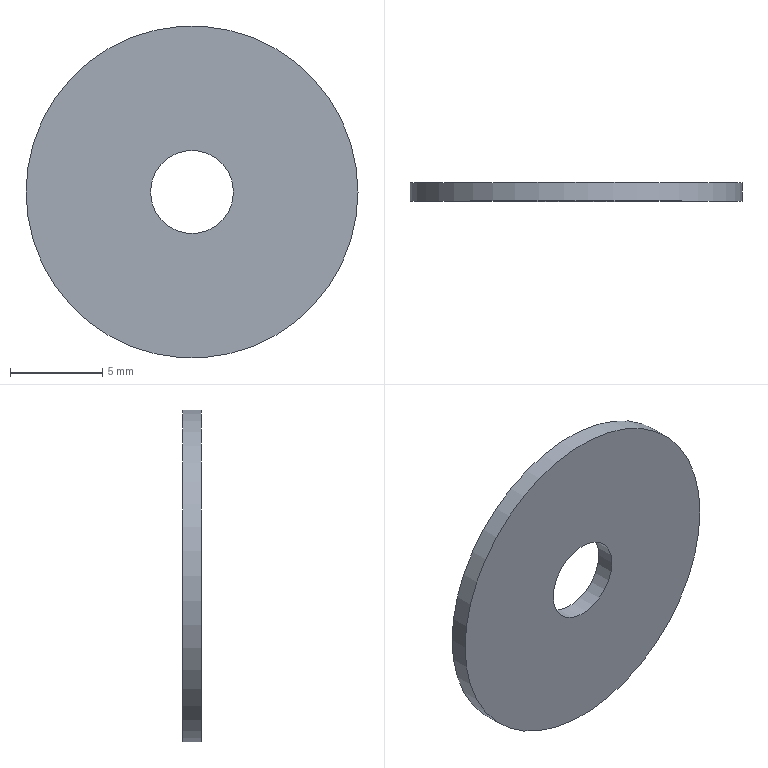Component | NX | 11 | 1 solid | 4 faces | box 18 x 1 x 18 mm | volume 239 mm3 | cylinder 2 | plane 2 | commonest cylinder face diameters 18 x1 4.5 x1
STEP:
#1=CARTESIAN_POINT('',(0.,0.,0.));
#2=DIRECTION('',(0.,0.,1.));
#3=DIRECTION('',(1.,0.,0.));
#4=AXIS2_PLACEMENT_3D('',#1,#2,#3);
#5=CARTESIAN_POINT('',(4.42,100.798,0.));
#6=VERTEX_POINT('',#5);
#7=CARTESIAN_POINT('',(-4.58,100.798,0.));
#8=DIRECTION('',(0.,-1.,0.));
#9=DIRECTION('',(1.,0.,-0.));
#10=AXIS2_PLACEMENT_3D('',#7,#8,#9);
#11=CIRCLE('',#10,9.);
#12=CARTESIAN_POINT('',(-4.58,100.798,0.));
#13=DIRECTION('',(0.,-1.,0.));
#14=DIRECTION('',(-1.,0.,0.));
#15=AXIS2_PLACEMENT_3D('',#12,#13,#14);
#16=CYLINDRICAL_SURFACE('',#15,9.);
#17=CARTESIAN_POINT('',(3.142,0.));
#18=DIRECTION('',(1.,0.));
#19=VECTOR('',#18,1.);
#20=LINE('',#17,#19);
#21=(GEOMETRIC_REPRESENTATION_CONTEXT(2)PARAMETRIC_REPRESENTATION_CONTEXT()REPRESENTATION_CONTEXT('',''));
#22=DEFINITIONAL_REPRESENTATION('',(#20),#21);
#23=PCURVE('',#16,#22);
#24=CARTESIAN_POINT('',(-4.58,100.798,0.));
#25=DIRECTION('',(0.,-1.,0.));
#26=DIRECTION('',(-1.,0.,0.));
#27=AXIS2_PLACEMENT_3D('',#24,#25,#26);
#28=PLANE('',#27);
#29=CARTESIAN_POINT('',(0.,0.));
#30=DIRECTION('',(-1.,0.));
#31=AXIS2_PLACEMENT_2D('',#29,#30);
#32=CIRCLE('',#31,9.);
#33=(GEOMETRIC_REPRESENTATION_CONTEXT(2)PARAMETRIC_REPRESENTATION_CONTEXT()REPRESENTATION_CONTEXT('',''));
#34=DEFINITIONAL_REPRESENTATION('',(#32),#33);
#35=PCURVE('',#28,#34);
#36=SURFACE_CURVE('',#11,(#23,#35),.PCURVE_S1.);
#37=EDGE_CURVE('',#6,#6,#36,.T.);
#38=ORIENTED_EDGE('',*,*,#37,.T.);
#39=CARTESIAN_POINT('',(4.42,99.798,0.));
#40=VERTEX_POINT('',#39);
#41=CARTESIAN_POINT('',(4.42,100.798,0.));
#42=CARTESIAN_POINT('',(4.42,99.798,0.));
#43=B_SPLINE_CURVE_WITH_KNOTS('',1,(#41,#42),.UNSPECIFIED.,.F.,.F.,(2,2),(0.,1.),.PIECEWISE_BEZIER_KNOTS.);
#44=CARTESIAN_POINT('',(9.425,0.));
#45=DIRECTION('',(0.,1.));
#46=VECTOR('',#45,1.);
#47=LINE('',#44,#46);
#48=(GEOMETRIC_REPRESENTATION_CONTEXT(2)PARAMETRIC_REPRESENTATION_CONTEXT()REPRESENTATION_CONTEXT('',''));
#49=DEFINITIONAL_REPRESENTATION('',(#47),#48);
#50=PCURVE('',#16,#49);
#51=CARTESIAN_POINT('',(3.142,0.));
#52=DIRECTION('',(0.,1.));
#53=VECTOR('',#52,1.);
#54=LINE('',#51,#53);
#55=(GEOMETRIC_REPRESENTATION_CONTEXT(2)PARAMETRIC_REPRESENTATION_CONTEXT()REPRESENTATION_CONTEXT('',''));
#56=DEFINITIONAL_REPRESENTATION('',(#54),#55);
#57=PCURVE('',#16,#56);
#58=SEAM_CURVE('',#43,(#50,#57),.PCURVE_S1.);
#59=EDGE_CURVE('',#6,#40,#58,.T.);
#60=ORIENTED_EDGE('',*,*,#59,.T.);
#61=CARTESIAN_POINT('',(-4.58,99.798,0.));
#62=DIRECTION('',(0.,-1.,0.));
#63=DIRECTION('',(1.,0.,-0.));
#64=AXIS2_PLACEMENT_3D('',#61,#62,#63);
#65=CIRCLE('',#64,9.);
#66=CARTESIAN_POINT('',(3.142,1.));
#67=DIRECTION('',(1.,0.));
#68=VECTOR('',#67,1.);
#69=LINE('',#66,#68);
#70=(GEOMETRIC_REPRESENTATION_CONTEXT(2)PARAMETRIC_REPRESENTATION_CONTEXT()REPRESENTATION_CONTEXT('',''));
#71=DEFINITIONAL_REPRESENTATION('',(#69),#70);
#72=PCURVE('',#16,#71);
#73=CARTESIAN_POINT('',(-4.58,99.798,0.));
#74=DIRECTION('',(0.,-1.,0.));
#75=DIRECTION('',(-1.,0.,0.));
#76=AXIS2_PLACEMENT_3D('',#73,#74,#75);
#77=PLANE('',#76);
#78=CARTESIAN_POINT('',(0.,0.));
#79=DIRECTION('',(-1.,0.));
#80=AXIS2_PLACEMENT_2D('',#78,#79);
#81=CIRCLE('',#80,9.);
#82=(GEOMETRIC_REPRESENTATION_CONTEXT(2)PARAMETRIC_REPRESENTATION_CONTEXT()REPRESENTATION_CONTEXT('',''));
#83=DEFINITIONAL_REPRESENTATION('',(#81),#82);
#84=PCURVE('',#77,#83);
#85=SURFACE_CURVE('',#65,(#72,#84),.PCURVE_S1.);
#86=EDGE_CURVE('',#40,#40,#85,.T.);
#87=ORIENTED_EDGE('',*,*,#86,.F.);
#88=ORIENTED_EDGE('',*,*,#59,.F.);
#89=EDGE_LOOP('',(#38,#60,#87,#88));
#90=FACE_BOUND('',#89,.T.);
#91=ADVANCED_FACE('',(#90),#16,.T.);
#92=CARTESIAN_POINT('',(-2.33,100.798,0.));
#93=VERTEX_POINT('',#92);
#94=CARTESIAN_POINT('',(-4.58,100.798,0.));
#95=DIRECTION('',(0.,-1.,0.));
#96=DIRECTION('',(1.,0.,-0.));
#97=AXIS2_PLACEMENT_3D('',#94,#95,#96);
#98=CIRCLE('',#97,2.25);
#99=CARTESIAN_POINT('',(-4.58,100.798,0.));
#100=DIRECTION('',(0.,-1.,0.));
#101=DIRECTION('',(-1.,0.,0.));
#102=AXIS2_PLACEMENT_3D('',#99,#100,#101);
#103=CYLINDRICAL_SURFACE('',#102,2.25);
#104=CARTESIAN_POINT('',(3.142,0.));
#105=DIRECTION('',(1.,0.));
#106=VECTOR('',#105,1.);
#107=LINE('',#104,#106);
#108=(GEOMETRIC_REPRESENTATION_CONTEXT(2)PARAMETRIC_REPRESENTATION_CONTEXT()REPRESENTATION_CONTEXT('',''));
#109=DEFINITIONAL_REPRESENTATION('',(#107),#108);
#110=PCURVE('',#103,#109);
#111=CARTESIAN_POINT('',(0.,0.));
#112=DIRECTION('',(-1.,0.));
#113=AXIS2_PLACEMENT_2D('',#111,#112);
#114=CIRCLE('',#113,2.25);
#115=(GEOMETRIC_REPRESENTATION_CONTEXT(2)PARAMETRIC_REPRESENTATION_CONTEXT()REPRESENTATION_CONTEXT('',''));
#116=DEFINITIONAL_REPRESENTATION('',(#114),#115);
#117=PCURVE('',#28,#116);
#118=SURFACE_CURVE('',#98,(#110,#117),.PCURVE_S1.);
#119=EDGE_CURVE('',#93,#93,#118,.T.);
#120=ORIENTED_EDGE('',*,*,#119,.T.);
#121=CARTESIAN_POINT('',(-2.33,99.798,0.));
#122=VERTEX_POINT('',#121);
#123=CARTESIAN_POINT('',(-2.33,100.798,0.));
#124=CARTESIAN_POINT('',(-2.33,99.798,0.));
#125=B_SPLINE_CURVE_WITH_KNOTS('',1,(#123,#124),.UNSPECIFIED.,.F.,.F.,(2,2),(0.,1.),.PIECEWISE_BEZIER_KNOTS.);
#126=CARTESIAN_POINT('',(9.425,0.));
#127=DIRECTION('',(0.,1.));
#128=VECTOR('',#127,1.);
#129=LINE('',#126,#128);
#130=(GEOMETRIC_REPRESENTATION_CONTEXT(2)PARAMETRIC_REPRESENTATION_CONTEXT()REPRESENTATION_CONTEXT('',''));
#131=DEFINITIONAL_REPRESENTATION('',(#129),#130);
#132=PCURVE('',#103,#131);
#133=CARTESIAN_POINT('',(3.142,0.));
#134=DIRECTION('',(0.,1.));
#135=VECTOR('',#134,1.);
#136=LINE('',#133,#135);
#137=(GEOMETRIC_REPRESENTATION_CONTEXT(2)PARAMETRIC_REPRESENTATION_CONTEXT()REPRESENTATION_CONTEXT('',''));
#138=DEFINITIONAL_REPRESENTATION('',(#136),#137);
#139=PCURVE('',#103,#138);
#140=SEAM_CURVE('',#125,(#132,#139),.PCURVE_S1.);
#141=EDGE_CURVE('',#93,#122,#140,.T.);
#142=ORIENTED_EDGE('',*,*,#141,.T.);
#143=CARTESIAN_POINT('',(-4.58,99.798,0.));
#144=DIRECTION('',(0.,-1.,0.));
#145=DIRECTION('',(1.,0.,-0.));
#146=AXIS2_PLACEMENT_3D('',#143,#144,#145);
#147=CIRCLE('',#146,2.25);
#148=CARTESIAN_POINT('',(3.142,1.));
#149=DIRECTION('',(1.,0.));
#150=VECTOR('',#149,1.);
#151=LINE('',#148,#150);
#152=(GEOMETRIC_REPRESENTATION_CONTEXT(2)PARAMETRIC_REPRESENTATION_CONTEXT()REPRESENTATION_CONTEXT('',''));
#153=DEFINITIONAL_REPRESENTATION('',(#151),#152);
#154=PCURVE('',#103,#153);
#155=CARTESIAN_POINT('',(0.,0.));
#156=DIRECTION('',(-1.,0.));
#157=AXIS2_PLACEMENT_2D('',#155,#156);
#158=CIRCLE('',#157,2.25);
#159=(GEOMETRIC_REPRESENTATION_CONTEXT(2)PARAMETRIC_REPRESENTATION_CONTEXT()REPRESENTATION_CONTEXT('',''));
#160=DEFINITIONAL_REPRESENTATION('',(#158),#159);
#161=PCURVE('',#77,#160);
#162=SURFACE_CURVE('',#147,(#154,#161),.PCURVE_S1.);
#163=EDGE_CURVE('',#122,#122,#162,.T.);
#164=ORIENTED_EDGE('',*,*,#163,.F.);
#165=ORIENTED_EDGE('',*,*,#141,.F.);
#166=EDGE_LOOP('',(#120,#142,#164,#165));
#167=FACE_BOUND('',#166,.F.);
#168=ADVANCED_FACE('',(#167),#103,.F.);
#169=ORIENTED_EDGE('',*,*,#37,.F.);
#170=EDGE_LOOP('',(#169));
#171=FACE_BOUND('',#170,.T.);
#172=ORIENTED_EDGE('',*,*,#119,.T.);
#173=EDGE_LOOP('',(#172));
#174=FACE_BOUND('',#173,.T.);
#175=ADVANCED_FACE('',(#171,#174),#28,.F.);
#176=ORIENTED_EDGE('',*,*,#86,.T.);
#177=EDGE_LOOP('',(#176));
#178=FACE_BOUND('',#177,.T.);
#179=ORIENTED_EDGE('',*,*,#163,.F.);
#180=EDGE_LOOP('',(#179));
#181=FACE_BOUND('',#180,.T.);
#182=ADVANCED_FACE('',(#178,#181),#77,.T.);
#183=CLOSED_SHELL('',(#91,#168,#175,#182));
#184=MANIFOLD_SOLID_BREP('',#183);
#185=(LENGTH_UNIT()NAMED_UNIT(*)SI_UNIT(.MILLI.,.METRE.));
#186=UNCERTAINTY_MEASURE_WITH_UNIT(LENGTH_MEASURE(0.00001),#185,'','');
#187=(NAMED_UNIT(*)PLANE_ANGLE_UNIT()SI_UNIT($,.RADIAN.));
#188=(NAMED_UNIT(*)SI_UNIT($,.STERADIAN.)SOLID_ANGLE_UNIT());
#189=(GEOMETRIC_REPRESENTATION_CONTEXT(3)GLOBAL_UNCERTAINTY_ASSIGNED_CONTEXT((#186))GLOBAL_UNIT_ASSIGNED_CONTEXT((#185,#187,#188))REPRESENTATION_CONTEXT('',''));
#190=ADVANCED_BREP_SHAPE_REPRESENTATION('',(#4,#184),#189);